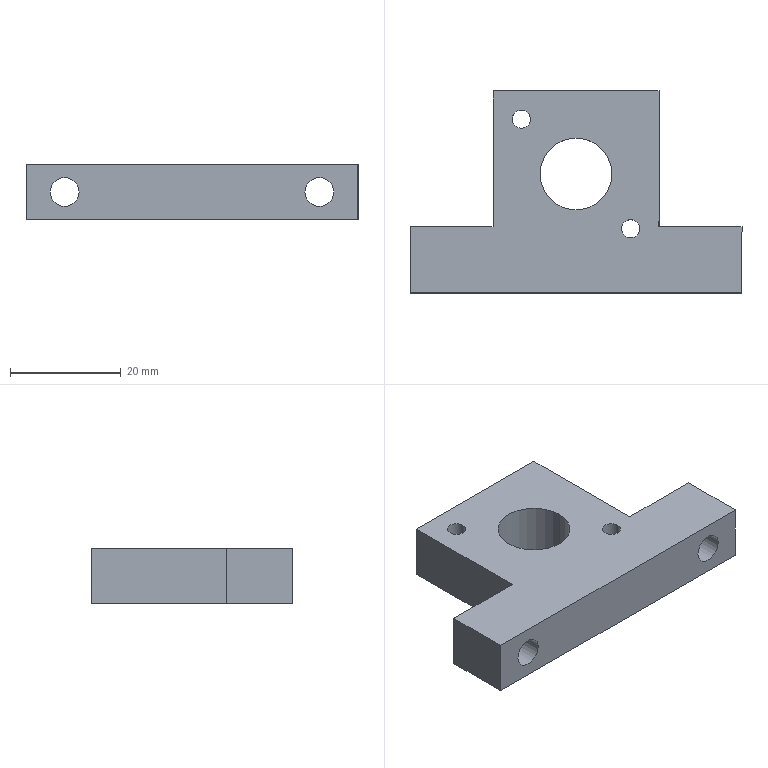Component | SolidWorks | AirCylinderSupportBlock2-1 | 1 solid | 20 faces | box 60 x 36.5 x 10 mm | volume 12542 mm3 | cylinder 10 | plane 10 | commonest cylinder face diameters 3.3 x4 5.2 x4 13 x2 | material 1023 Carbon Steel Plate (SS)
build123d program:
from build123d import *

# Parameters (mm, degrees)
SKETCH1_R                  = 6.5
BOSS_EXTRUDE1_DEPTH        = 10
F_5_2_5_2_DIAMETER_HOLE1_D = 5.2
M4_TAPPED_HOLE1_D          = 3.3
M4_TAPPED_HOLE1_DEPTH      = 11.5
M4_TAPPED_HOLE1_TIP        = 0.9914


with BuildPart() as part:
    # Sketch1 → Boss-Extrude1 (new body)
    with BuildSketch(Plane(origin=(0, 0, 0), x_dir=(0, 0, -1), z_dir=(1, 0, 0))):
        Polygon((73.374, 68.957), (73.374, 44.457), (88.374, 44.457), (88.374, 32.457), (28.374, 32.457), (28.374, 44.457), (43.374, 44.457), (43.374, 68.957), align=None)
        with Locations((58.374, 53.957)):
            Circle(SKETCH1_R, mode=Mode.SUBTRACT)
    extrude(amount=BOSS_EXTRUDE1_DEPTH)

    # 5.2 _5.2_ Diameter Hole1 (through all)
    with Locations(Plane(origin=(0, 44.457, 0), x_dir=(-1, 0, 0), z_dir=(0, 1, 0))):
        with Locations((-5, -35.374), (-5, -81.374)):
            Hole(F_5_2_5_2_DIAMETER_HOLE1_D / 2)

    # M4 Tapped Hole1
    with Locations(Plane(origin=(10, 0, 0), x_dir=(0, 0, -1), z_dir=(1, 0, 0))):
        with Locations((68.274, 63.857), (48.474, 44.057)):
            Hole(M4_TAPPED_HOLE1_D / 2, depth=M4_TAPPED_HOLE1_DEPTH)
            with Locations((0, 0, -(M4_TAPPED_HOLE1_DEPTH + M4_TAPPED_HOLE1_TIP / 2))):  # 118° drill point
                Cone(0, M4_TAPPED_HOLE1_D / 2, M4_TAPPED_HOLE1_TIP, mode=Mode.SUBTRACT)


solid = part.part

# Placed as in the assembly
solid = solid.moved(Location((51.459, -33.763, 34.579), (0, 90, 0)))
STEP:
#1=CARTESIAN_POINT('',(-0.727,1.185,1.361));
#2=VERTEX_POINT('',#1);
#3=CARTESIAN_POINT('',(-0.5971,1.185,1.361));
#4=VERTEX_POINT('',#3);
#5=CARTESIAN_POINT('',(-0.662,1.185,1.361));
#6=DIRECTION('',(-0.,-0.,1.));
#7=DIRECTION('',(1.,-0.,0.));
#8=AXIS2_PLACEMENT_3D('',#5,#6,#7);
#9=CIRCLE('',#8,0.06496);
#10=EDGE_CURVE('',#2,#4,#9,.T.);
#11=ORIENTED_EDGE('',*,*,#10,.T.);
#12=CARTESIAN_POINT('',(-0.5971,1.185,0.9677));
#13=VERTEX_POINT('',#12);
#14=CARTESIAN_POINT('',(-0.5971,1.185,0.9677));
#15=DIRECTION('',(0.,0.,-1.));
#16=VECTOR('',#15,39.37);
#17=LINE('',#14,#16);
#18=EDGE_CURVE('',#4,#13,#17,.T.);
#19=ORIENTED_EDGE('',*,*,#18,.T.);
#20=CARTESIAN_POINT('',(-0.727,1.185,0.9677));
#21=VERTEX_POINT('',#20);
#22=CARTESIAN_POINT('',(-0.662,1.185,0.9677));
#23=DIRECTION('',(0.,0.,-1.));
#24=DIRECTION('',(-1.,0.,0.));
#25=AXIS2_PLACEMENT_3D('',#22,#23,#24);
#26=CIRCLE('',#25,0.06496);
#27=EDGE_CURVE('',#13,#21,#26,.T.);
#28=ORIENTED_EDGE('',*,*,#27,.T.);
#29=CARTESIAN_POINT('',(-0.727,1.185,0.9677));
#30=DIRECTION('',(0.,0.,-1.));
#31=VECTOR('',#30,39.37);
#32=LINE('',#29,#31);
#33=EDGE_CURVE('',#2,#21,#32,.T.);
#34=ORIENTED_EDGE('',*,*,#33,.F.);
#35=EDGE_LOOP('',(#11,#19,#28,#34));
#36=FACE_OUTER_BOUND('',#35,.T.);
#37=CARTESIAN_POINT('',(-0.662,1.185,0.9677));
#38=DIRECTION('',(0.,0.,-1.));
#39=DIRECTION('',(-1.,0.,0.));
#40=AXIS2_PLACEMENT_3D('',#37,#38,#39);
#41=CYLINDRICAL_SURFACE('',#40,0.06496);
#42=ADVANCED_FACE('',(#36),#41,.F.);
#43=CARTESIAN_POINT('',(0.05256,0.4053,1.361));
#44=VERTEX_POINT('',#43);
#45=CARTESIAN_POINT('',(0.1825,0.4053,1.361));
#46=VERTEX_POINT('',#45);
#47=CARTESIAN_POINT('',(0.1175,0.4053,1.361));
#48=DIRECTION('',(-0.,-0.,1.));
#49=DIRECTION('',(1.,-0.,0.));
#50=AXIS2_PLACEMENT_3D('',#47,#48,#49);
#51=CIRCLE('',#50,0.06496);
#52=EDGE_CURVE('',#44,#46,#51,.T.);
#53=ORIENTED_EDGE('',*,*,#52,.T.);
#54=CARTESIAN_POINT('',(0.1825,0.4053,0.9677));
#55=VERTEX_POINT('',#54);
#56=CARTESIAN_POINT('',(0.1825,0.4053,0.9677));
#57=DIRECTION('',(0.,0.,-1.));
#58=VECTOR('',#57,39.37);
#59=LINE('',#56,#58);
#60=EDGE_CURVE('',#46,#55,#59,.T.);
#61=ORIENTED_EDGE('',*,*,#60,.T.);
#62=CARTESIAN_POINT('',(0.05256,0.4053,0.9677));
#63=VERTEX_POINT('',#62);
#64=CARTESIAN_POINT('',(0.1175,0.4053,0.9677));
#65=DIRECTION('',(0.,0.,-1.));
#66=DIRECTION('',(-1.,0.,0.));
#67=AXIS2_PLACEMENT_3D('',#64,#65,#66);
#68=CIRCLE('',#67,0.06496);
#69=EDGE_CURVE('',#55,#63,#68,.T.);
#70=ORIENTED_EDGE('',*,*,#69,.T.);
#71=CARTESIAN_POINT('',(0.05256,0.4053,0.9677));
#72=DIRECTION('',(0.,0.,-1.));
#73=VECTOR('',#72,39.37);
#74=LINE('',#71,#73);
#75=EDGE_CURVE('',#44,#63,#74,.T.);
#76=ORIENTED_EDGE('',*,*,#75,.F.);
#77=EDGE_LOOP('',(#53,#61,#70,#76));
#78=FACE_OUTER_BOUND('',#77,.T.);
#79=CARTESIAN_POINT('',(0.1175,0.4053,0.9677));
#80=DIRECTION('',(0.,0.,-1.));
#81=DIRECTION('',(-1.,0.,0.));
#82=AXIS2_PLACEMENT_3D('',#79,#80,#81);
#83=CYLINDRICAL_SURFACE('',#82,0.06496);
#84=ADVANCED_FACE('',(#78),#83,.F.);
#85=CARTESIAN_POINT('',(0.5309,-0.05139,1.165));
#86=VERTEX_POINT('',#85);
#87=CARTESIAN_POINT('',(0.7356,-0.05139,1.165));
#88=VERTEX_POINT('',#87);
#89=CARTESIAN_POINT('',(0.6333,-0.05139,1.165));
#90=DIRECTION('',(0.,1.,0.));
#91=DIRECTION('',(1.,-0.,0.));
#92=AXIS2_PLACEMENT_3D('',#89,#90,#91);
#93=CIRCLE('',#92,0.1024);
#94=EDGE_CURVE('',#86,#88,#93,.T.);
#95=ORIENTED_EDGE('',*,*,#94,.F.);
#96=CARTESIAN_POINT('',(0.5309,0.421,1.165));
#97=VERTEX_POINT('',#96);
#98=CARTESIAN_POINT('',(0.5309,0.421,1.165));
#99=DIRECTION('',(0.,1.,0.));
#100=VECTOR('',#99,39.37);
#101=LINE('',#98,#100);
#102=EDGE_CURVE('',#86,#97,#101,.T.);
#103=ORIENTED_EDGE('',*,*,#102,.T.);
#104=CARTESIAN_POINT('',(0.7356,0.421,1.165));
#105=VERTEX_POINT('',#104);
#106=CARTESIAN_POINT('',(0.6333,0.421,1.165));
#107=DIRECTION('',(0.,1.,0.));
#108=DIRECTION('',(1.,-0.,0.));
#109=AXIS2_PLACEMENT_3D('',#106,#107,#108);
#110=CIRCLE('',#109,0.1024);
#111=EDGE_CURVE('',#97,#105,#110,.T.);
#112=ORIENTED_EDGE('',*,*,#111,.T.);
#113=CARTESIAN_POINT('',(0.7356,0.421,1.165));
#114=DIRECTION('',(0.,1.,0.));
#115=VECTOR('',#114,39.37);
#116=LINE('',#113,#115);
#117=EDGE_CURVE('',#88,#105,#116,.T.);
#118=ORIENTED_EDGE('',*,*,#117,.F.);
#119=EDGE_LOOP('',(#95,#103,#112,#118));
#120=FACE_OUTER_BOUND('',#119,.T.);
#121=CARTESIAN_POINT('',(0.6333,0.421,1.165));
#122=DIRECTION('',(0.,1.,0.));
#123=DIRECTION('',(1.,-0.,0.));
#124=AXIS2_PLACEMENT_3D('',#121,#122,#123);
#125=CYLINDRICAL_SURFACE('',#124,0.1024);
#126=ADVANCED_FACE('',(#120),#125,.F.);
#127=CARTESIAN_POINT('',(-1.28,-0.05139,1.165));
#128=VERTEX_POINT('',#127);
#129=CARTESIAN_POINT('',(-1.075,-0.05139,1.165));
#130=VERTEX_POINT('',#129);
#131=CARTESIAN_POINT('',(-1.178,-0.05139,1.165));
#132=DIRECTION('',(0.,1.,0.));
#133=DIRECTION('',(1.,-0.,0.));
#134=AXIS2_PLACEMENT_3D('',#131,#132,#133);
#135=CIRCLE('',#134,0.1024);
#136=EDGE_CURVE('',#128,#130,#135,.T.);
#137=ORIENTED_EDGE('',*,*,#136,.F.);
#138=CARTESIAN_POINT('',(-1.28,0.421,1.165));
#139=VERTEX_POINT('',#138);
#140=CARTESIAN_POINT('',(-1.28,0.421,1.165));
#141=DIRECTION('',(0.,1.,0.));
#142=VECTOR('',#141,39.37);
#143=LINE('',#140,#142);
#144=EDGE_CURVE('',#128,#139,#143,.T.);
#145=ORIENTED_EDGE('',*,*,#144,.T.);
#146=CARTESIAN_POINT('',(-1.075,0.421,1.165));
#147=VERTEX_POINT('',#146);
#148=CARTESIAN_POINT('',(-1.178,0.421,1.165));
#149=DIRECTION('',(0.,1.,0.));
#150=DIRECTION('',(1.,-0.,0.));
#151=AXIS2_PLACEMENT_3D('',#148,#149,#150);
#152=CIRCLE('',#151,0.1024);
#153=EDGE_CURVE('',#139,#147,#152,.T.);
#154=ORIENTED_EDGE('',*,*,#153,.T.);
#155=CARTESIAN_POINT('',(-1.075,0.421,1.165));
#156=DIRECTION('',(0.,1.,0.));
#157=VECTOR('',#156,39.37);
#158=LINE('',#155,#157);
#159=EDGE_CURVE('',#130,#147,#158,.T.);
#160=ORIENTED_EDGE('',*,*,#159,.F.);
#161=EDGE_LOOP('',(#137,#145,#154,#160));
#162=FACE_OUTER_BOUND('',#161,.T.);
#163=CARTESIAN_POINT('',(-1.178,0.421,1.165));
#164=DIRECTION('',(0.,1.,0.));
#165=DIRECTION('',(1.,-0.,0.));
#166=AXIS2_PLACEMENT_3D('',#163,#164,#165);
#167=CYLINDRICAL_SURFACE('',#166,0.1024);
#168=ADVANCED_FACE('',(#162),#167,.F.);
#169=CARTESIAN_POINT('',(-0.01634,0.7951,0.9677));
#170=VERTEX_POINT('',#169);
#171=CARTESIAN_POINT('',(-0.5282,0.7951,0.9677));
#172=VERTEX_POINT('',#171);
#173=CARTESIAN_POINT('',(-0.2722,0.7951,0.9677));
#174=DIRECTION('',(0.,0.,-1.));
#175=DIRECTION('',(-1.,0.,0.));
#176=AXIS2_PLACEMENT_3D('',#173,#174,#175);
#177=CIRCLE('',#176,0.2559);
#178=EDGE_CURVE('',#170,#172,#177,.T.);
#179=ORIENTED_EDGE('',*,*,#178,.T.);
#180=CARTESIAN_POINT('',(-0.5282,0.7951,1.361));
#181=VERTEX_POINT('',#180);
#182=CARTESIAN_POINT('',(-0.5282,0.7951,0.9677));
#183=DIRECTION('',(-0.,-0.,1.));
#184=VECTOR('',#183,39.37);
#185=LINE('',#182,#184);
#186=EDGE_CURVE('',#172,#181,#185,.T.);
#187=ORIENTED_EDGE('',*,*,#186,.T.);
#188=CARTESIAN_POINT('',(-0.01634,0.7951,1.361));
#189=VERTEX_POINT('',#188);
#190=CARTESIAN_POINT('',(-0.2722,0.7951,1.361));
#191=DIRECTION('',(0.,0.,-1.));
#192=DIRECTION('',(-1.,0.,0.));
#193=AXIS2_PLACEMENT_3D('',#190,#191,#192);
#194=CIRCLE('',#193,0.2559);
#195=EDGE_CURVE('',#189,#181,#194,.T.);
#196=ORIENTED_EDGE('',*,*,#195,.F.);
#197=CARTESIAN_POINT('',(-0.01634,0.7951,0.9677));
#198=DIRECTION('',(-0.,-0.,1.));
#199=VECTOR('',#198,39.37);
#200=LINE('',#197,#199);
#201=EDGE_CURVE('',#170,#189,#200,.T.);
#202=ORIENTED_EDGE('',*,*,#201,.F.);
#203=EDGE_LOOP('',(#179,#187,#196,#202));
#204=FACE_OUTER_BOUND('',#203,.T.);
#205=CARTESIAN_POINT('',(-0.2722,0.7951,0.9677));
#206=DIRECTION('',(-0.,-0.,1.));
#207=DIRECTION('',(1.,-0.,0.));
#208=AXIS2_PLACEMENT_3D('',#205,#206,#207);
#209=CYLINDRICAL_SURFACE('',#208,0.2559);
#210=ADVANCED_FACE('',(#204),#209,.F.);
#211=CARTESIAN_POINT('',(-0.662,1.185,0.9677));
#212=DIRECTION('',(0.,0.,-1.));
#213=DIRECTION('',(-1.,0.,0.));
#214=AXIS2_PLACEMENT_3D('',#211,#212,#213);
#215=CIRCLE('',#214,0.06496);
#216=EDGE_CURVE('',#21,#13,#215,.T.);
#217=ORIENTED_EDGE('',*,*,#216,.F.);
#218=ORIENTED_EDGE('',*,*,#27,.F.);
#219=EDGE_LOOP('',(#217,#218));
#220=FACE_BOUND('',#219,.T.);
#221=CARTESIAN_POINT('',(0.1175,0.4053,0.9677));
#222=DIRECTION('',(0.,0.,-1.));
#223=DIRECTION('',(-1.,0.,0.));
#224=AXIS2_PLACEMENT_3D('',#221,#222,#223);
#225=CIRCLE('',#224,0.06496);
#226=EDGE_CURVE('',#63,#55,#225,.T.);
#227=ORIENTED_EDGE('',*,*,#226,.F.);
#228=ORIENTED_EDGE('',*,*,#69,.F.);
#229=EDGE_LOOP('',(#227,#228));
#230=FACE_BOUND('',#229,.T.);
#231=CARTESIAN_POINT('',(-0.8628,1.386,0.9677));
#232=VERTEX_POINT('',#231);
#233=CARTESIAN_POINT('',(0.3183,1.386,0.9677));
#234=VERTEX_POINT('',#233);
#235=CARTESIAN_POINT('',(0.3183,1.386,0.9677));
#236=DIRECTION('',(1.,-0.,0.));
#237=VECTOR('',#236,39.37);
#238=LINE('',#235,#237);
#239=EDGE_CURVE('',#232,#234,#238,.T.);
#240=ORIENTED_EDGE('',*,*,#239,.T.);
#241=CARTESIAN_POINT('',(0.3183,0.421,0.9677));
#242=VERTEX_POINT('',#241);
#243=CARTESIAN_POINT('',(0.3183,1.386,0.9677));
#244=DIRECTION('',(-0.,-1.,-0.));
#245=VECTOR('',#244,39.37);
#246=LINE('',#243,#245);
#247=EDGE_CURVE('',#234,#242,#246,.T.);
#248=ORIENTED_EDGE('',*,*,#247,.T.);
#249=CARTESIAN_POINT('',(0.9089,0.421,0.9677));
#250=VERTEX_POINT('',#249);
#251=CARTESIAN_POINT('',(0.9089,0.421,0.9677));
#252=DIRECTION('',(1.,-0.,0.));
#253=VECTOR('',#252,39.37);
#254=LINE('',#251,#253);
#255=EDGE_CURVE('',#242,#250,#254,.T.);
#256=ORIENTED_EDGE('',*,*,#255,.T.);
#257=CARTESIAN_POINT('',(0.9089,-0.05139,0.9677));
#258=VERTEX_POINT('',#257);
#259=CARTESIAN_POINT('',(0.9089,-0.05139,0.9677));
#260=DIRECTION('',(-0.,-1.,-0.));
#261=VECTOR('',#260,39.37);
#262=LINE('',#259,#261);
#263=EDGE_CURVE('',#250,#258,#262,.T.);
#264=ORIENTED_EDGE('',*,*,#263,.T.);
#265=CARTESIAN_POINT('',(-1.453,-0.05139,0.9677));
#266=VERTEX_POINT('',#265);
#267=CARTESIAN_POINT('',(-1.453,-0.05139,0.9677));
#268=DIRECTION('',(-1.,0.,-0.));
#269=VECTOR('',#268,39.37);
#270=LINE('',#267,#269);
#271=EDGE_CURVE('',#258,#266,#270,.T.);
#272=ORIENTED_EDGE('',*,*,#271,.T.);
#273=CARTESIAN_POINT('',(-1.453,0.421,0.9677));
#274=VERTEX_POINT('',#273);
#275=CARTESIAN_POINT('',(-1.453,0.421,0.9677));
#276=DIRECTION('',(0.,1.,0.));
#277=VECTOR('',#276,39.37);
#278=LINE('',#275,#277);
#279=EDGE_CURVE('',#266,#274,#278,.T.);
#280=ORIENTED_EDGE('',*,*,#279,.T.);
#281=CARTESIAN_POINT('',(-0.8628,0.421,0.9677));
#282=VERTEX_POINT('',#281);
#283=CARTESIAN_POINT('',(-0.8628,0.421,0.9677));
#284=DIRECTION('',(1.,-0.,0.));
#285=VECTOR('',#284,39.37);
#286=LINE('',#283,#285);
#287=EDGE_CURVE('',#274,#282,#286,.T.);
#288=ORIENTED_EDGE('',*,*,#287,.T.);
#289=CARTESIAN_POINT('',(-0.8628,1.386,0.9677));
#290=DIRECTION('',(0.,1.,0.));
#291=VECTOR('',#290,39.37);
#292=LINE('',#289,#291);
#293=EDGE_CURVE('',#282,#232,#292,.T.);
#294=ORIENTED_EDGE('',*,*,#293,.T.);
#295=EDGE_LOOP('',(#240,#248,#256,#264,#272,#280,#288,#294));
#296=FACE_OUTER_BOUND('',#295,.T.);
#297=ORIENTED_EDGE('',*,*,#178,.F.);
#298=CARTESIAN_POINT('',(-0.2722,0.7951,0.9677));
#299=DIRECTION('',(0.,0.,-1.));
#300=DIRECTION('',(-1.,0.,0.));
#301=AXIS2_PLACEMENT_3D('',#298,#299,#300);
#302=CIRCLE('',#301,0.2559);
#303=EDGE_CURVE('',#172,#170,#302,.T.);
#304=ORIENTED_EDGE('',*,*,#303,.F.);
#305=EDGE_LOOP('',(#297,#304));
#306=FACE_BOUND('',#305,.T.);
#307=CARTESIAN_POINT('',(-0.8628,1.386,0.9677));
#308=DIRECTION('',(-0.,-0.,1.));
#309=DIRECTION('',(1.,-0.,0.));
#310=AXIS2_PLACEMENT_3D('',#307,#308,#309);
#311=PLANE('',#310);
#312=ADVANCED_FACE('',(#220,#230,#296,#306),#311,.F.);
#313=ORIENTED_EDGE('',*,*,#10,.F.);
#314=CARTESIAN_POINT('',(-0.662,1.185,1.361));
#315=DIRECTION('',(-0.,-0.,1.));
#316=DIRECTION('',(1.,-0.,0.));
#317=AXIS2_PLACEMENT_3D('',#314,#315,#316);
#318=CIRCLE('',#317,0.06496);
#319=EDGE_CURVE('',#4,#2,#318,.T.);
#320=ORIENTED_EDGE('',*,*,#319,.F.);
#321=EDGE_LOOP('',(#313,#320));
#322=FACE_BOUND('',#321,.T.);
#323=ORIENTED_EDGE('',*,*,#52,.F.);
#324=CARTESIAN_POINT('',(0.1175,0.4053,1.361));
#325=DIRECTION('',(-0.,-0.,1.));
#326=DIRECTION('',(1.,-0.,0.));
#327=AXIS2_PLACEMENT_3D('',#324,#325,#326);
#328=CIRCLE('',#327,0.06496);
#329=EDGE_CURVE('',#46,#44,#328,.T.);
#330=ORIENTED_EDGE('',*,*,#329,.F.);
#331=EDGE_LOOP('',(#323,#330));
#332=FACE_BOUND('',#331,.T.);
#333=CARTESIAN_POINT('',(-0.8628,1.386,1.361));
#334=VERTEX_POINT('',#333);
#335=CARTESIAN_POINT('',(0.3183,1.386,1.361));
#336=VERTEX_POINT('',#335);
#337=CARTESIAN_POINT('',(0.3183,1.386,1.361));
#338=DIRECTION('',(1.,-0.,0.));
#339=VECTOR('',#338,39.37);
#340=LINE('',#337,#339);
#341=EDGE_CURVE('',#334,#336,#340,.T.);
#342=ORIENTED_EDGE('',*,*,#341,.F.);
#343=CARTESIAN_POINT('',(-0.8628,0.421,1.361));
#344=VERTEX_POINT('',#343);
#345=CARTESIAN_POINT('',(-0.8628,1.386,1.361));
#346=DIRECTION('',(0.,1.,0.));
#347=VECTOR('',#346,39.37);
#348=LINE('',#345,#347);
#349=EDGE_CURVE('',#344,#334,#348,.T.);
#350=ORIENTED_EDGE('',*,*,#349,.F.);
#351=CARTESIAN_POINT('',(-1.453,0.421,1.361));
#352=VERTEX_POINT('',#351);
#353=CARTESIAN_POINT('',(-0.8628,0.421,1.361));
#354=DIRECTION('',(1.,-0.,0.));
#355=VECTOR('',#354,39.37);
#356=LINE('',#353,#355);
#357=EDGE_CURVE('',#352,#344,#356,.T.);
#358=ORIENTED_EDGE('',*,*,#357,.F.);
#359=CARTESIAN_POINT('',(-1.453,-0.05139,1.361));
#360=VERTEX_POINT('',#359);
#361=CARTESIAN_POINT('',(-1.453,0.421,1.361));
#362=DIRECTION('',(0.,1.,0.));
#363=VECTOR('',#362,39.37);
#364=LINE('',#361,#363);
#365=EDGE_CURVE('',#360,#352,#364,.T.);
#366=ORIENTED_EDGE('',*,*,#365,.F.);
#367=CARTESIAN_POINT('',(0.9089,-0.05139,1.361));
#368=VERTEX_POINT('',#367);
#369=CARTESIAN_POINT('',(-1.453,-0.05139,1.361));
#370=DIRECTION('',(-1.,0.,-0.));
#371=VECTOR('',#370,39.37);
#372=LINE('',#369,#371);
#373=EDGE_CURVE('',#368,#360,#372,.T.);
#374=ORIENTED_EDGE('',*,*,#373,.F.);
#375=CARTESIAN_POINT('',(0.9089,0.421,1.361));
#376=VERTEX_POINT('',#375);
#377=CARTESIAN_POINT('',(0.9089,-0.05139,1.361));
#378=DIRECTION('',(-0.,-1.,-0.));
#379=VECTOR('',#378,39.37);
#380=LINE('',#377,#379);
#381=EDGE_CURVE('',#376,#368,#380,.T.);
#382=ORIENTED_EDGE('',*,*,#381,.F.);
#383=CARTESIAN_POINT('',(0.3183,0.421,1.361));
#384=VERTEX_POINT('',#383);
#385=CARTESIAN_POINT('',(0.9089,0.421,1.361));
#386=DIRECTION('',(1.,-0.,0.));
#387=VECTOR('',#386,39.37);
#388=LINE('',#385,#387);
#389=EDGE_CURVE('',#384,#376,#388,.T.);
#390=ORIENTED_EDGE('',*,*,#389,.F.);
#391=CARTESIAN_POINT('',(0.3183,1.386,1.361));
#392=DIRECTION('',(-0.,-1.,-0.));
#393=VECTOR('',#392,39.37);
#394=LINE('',#391,#393);
#395=EDGE_CURVE('',#336,#384,#394,.T.);
#396=ORIENTED_EDGE('',*,*,#395,.F.);
#397=EDGE_LOOP('',(#342,#350,#358,#366,#374,#382,#390,#396));
#398=FACE_OUTER_BOUND('',#397,.T.);
#399=ORIENTED_EDGE('',*,*,#195,.T.);
#400=CARTESIAN_POINT('',(-0.2722,0.7951,1.361));
#401=DIRECTION('',(0.,0.,-1.));
#402=DIRECTION('',(-1.,0.,0.));
#403=AXIS2_PLACEMENT_3D('',#400,#401,#402);
#404=CIRCLE('',#403,0.2559);
#405=EDGE_CURVE('',#181,#189,#404,.T.);
#406=ORIENTED_EDGE('',*,*,#405,.T.);
#407=EDGE_LOOP('',(#399,#406));
#408=FACE_BOUND('',#407,.T.);
#409=CARTESIAN_POINT('',(-0.8628,1.386,1.361));
#410=DIRECTION('',(-0.,-0.,1.));
#411=DIRECTION('',(1.,-0.,0.));
#412=AXIS2_PLACEMENT_3D('',#409,#410,#411);
#413=PLANE('',#412);
#414=ADVANCED_FACE('',(#322,#332,#398,#408),#413,.T.);
#415=ORIENTED_EDGE('',*,*,#341,.T.);
#416=CARTESIAN_POINT('',(0.3183,1.386,0.9677));
#417=DIRECTION('',(-0.,-0.,1.));
#418=VECTOR('',#417,39.37);
#419=LINE('',#416,#418);
#420=EDGE_CURVE('',#234,#336,#419,.T.);
#421=ORIENTED_EDGE('',*,*,#420,.F.);
#422=ORIENTED_EDGE('',*,*,#239,.F.);
#423=CARTESIAN_POINT('',(-0.8628,1.386,0.9677));
#424=DIRECTION('',(-0.,-0.,1.));
#425=VECTOR('',#424,39.37);
#426=LINE('',#423,#425);
#427=EDGE_CURVE('',#232,#334,#426,.T.);
#428=ORIENTED_EDGE('',*,*,#427,.T.);
#429=EDGE_LOOP('',(#415,#421,#422,#428));
#430=FACE_OUTER_BOUND('',#429,.T.);
#431=CARTESIAN_POINT('',(0.3183,1.386,0.9677));
#432=DIRECTION('',(-0.,-1.,-0.));
#433=DIRECTION('',(-1.,0.,-0.));
#434=AXIS2_PLACEMENT_3D('',#431,#432,#433);
#435=PLANE('',#434);
#436=ADVANCED_FACE('',(#430),#435,.F.);
#437=ORIENTED_EDGE('',*,*,#395,.T.);
#438=CARTESIAN_POINT('',(0.3183,0.421,0.9677));
#439=DIRECTION('',(-0.,-0.,1.));
#440=VECTOR('',#439,39.37);
#441=LINE('',#438,#440);
#442=EDGE_CURVE('',#242,#384,#441,.T.);
#443=ORIENTED_EDGE('',*,*,#442,.F.);
#444=ORIENTED_EDGE('',*,*,#247,.F.);
#445=ORIENTED_EDGE('',*,*,#420,.T.);
#446=EDGE_LOOP('',(#437,#443,#444,#445));
#447=FACE_OUTER_BOUND('',#446,.T.);
#448=CARTESIAN_POINT('',(0.3183,1.386,0.9677));
#449=DIRECTION('',(-1.,0.,-0.));
#450=DIRECTION('',(0.,1.,0.));
#451=AXIS2_PLACEMENT_3D('',#448,#449,#450);
#452=PLANE('',#451);
#453=ADVANCED_FACE('',(#447),#452,.F.);
#454=CARTESIAN_POINT('',(0.6333,0.421,1.165));
#455=DIRECTION('',(0.,1.,0.));
#456=DIRECTION('',(1.,-0.,0.));
#457=AXIS2_PLACEMENT_3D('',#454,#455,#456);
#458=CIRCLE('',#457,0.1024);
#459=EDGE_CURVE('',#105,#97,#458,.T.);
#460=ORIENTED_EDGE('',*,*,#459,.F.);
#461=ORIENTED_EDGE('',*,*,#111,.F.);
#462=EDGE_LOOP('',(#460,#461));
#463=FACE_BOUND('',#462,.T.);
#464=ORIENTED_EDGE('',*,*,#389,.T.);
#465=CARTESIAN_POINT('',(0.9089,0.421,0.9677));
#466=DIRECTION('',(-0.,-0.,1.));
#467=VECTOR('',#466,39.37);
#468=LINE('',#465,#467);
#469=EDGE_CURVE('',#250,#376,#468,.T.);
#470=ORIENTED_EDGE('',*,*,#469,.F.);
#471=ORIENTED_EDGE('',*,*,#255,.F.);
#472=ORIENTED_EDGE('',*,*,#442,.T.);
#473=EDGE_LOOP('',(#464,#470,#471,#472));
#474=FACE_OUTER_BOUND('',#473,.T.);
#475=CARTESIAN_POINT('',(0.9089,0.421,0.9677));
#476=DIRECTION('',(-0.,-1.,-0.));
#477=DIRECTION('',(-1.,0.,-0.));
#478=AXIS2_PLACEMENT_3D('',#475,#476,#477);
#479=PLANE('',#478);
#480=ADVANCED_FACE('',(#463,#474),#479,.F.);
#481=ORIENTED_EDGE('',*,*,#381,.T.);
#482=CARTESIAN_POINT('',(0.9089,-0.05139,0.9677));
#483=DIRECTION('',(-0.,-0.,1.));
#484=VECTOR('',#483,39.37);
#485=LINE('',#482,#484);
#486=EDGE_CURVE('',#258,#368,#485,.T.);
#487=ORIENTED_EDGE('',*,*,#486,.F.);
#488=ORIENTED_EDGE('',*,*,#263,.F.);
#489=ORIENTED_EDGE('',*,*,#469,.T.);
#490=EDGE_LOOP('',(#481,#487,#488,#489));
#491=FACE_OUTER_BOUND('',#490,.T.);
#492=CARTESIAN_POINT('',(0.9089,-0.05139,0.9677));
#493=DIRECTION('',(-1.,0.,-0.));
#494=DIRECTION('',(-0.,-0.,1.));
#495=AXIS2_PLACEMENT_3D('',#492,#493,#494);
#496=PLANE('',#495);
#497=ADVANCED_FACE('',(#491),#496,.F.);
#498=CARTESIAN_POINT('',(0.6333,-0.05139,1.165));
#499=DIRECTION('',(0.,1.,0.));
#500=DIRECTION('',(1.,-0.,0.));
#501=AXIS2_PLACEMENT_3D('',#498,#499,#500);
#502=CIRCLE('',#501,0.1024);
#503=EDGE_CURVE('',#88,#86,#502,.T.);
#504=ORIENTED_EDGE('',*,*,#503,.T.);
#505=ORIENTED_EDGE('',*,*,#94,.T.);
#506=EDGE_LOOP('',(#504,#505));
#507=FACE_BOUND('',#506,.T.);
#508=CARTESIAN_POINT('',(-1.178,-0.05139,1.165));
#509=DIRECTION('',(0.,1.,0.));
#510=DIRECTION('',(1.,-0.,0.));
#511=AXIS2_PLACEMENT_3D('',#508,#509,#510);
#512=CIRCLE('',#511,0.1024);
#513=EDGE_CURVE('',#130,#128,#512,.T.);
#514=ORIENTED_EDGE('',*,*,#513,.T.);
#515=ORIENTED_EDGE('',*,*,#136,.T.);
#516=EDGE_LOOP('',(#514,#515));
#517=FACE_BOUND('',#516,.T.);
#518=ORIENTED_EDGE('',*,*,#373,.T.);
#519=CARTESIAN_POINT('',(-1.453,-0.05139,0.9677));
#520=DIRECTION('',(-0.,-0.,1.));
#521=VECTOR('',#520,39.37);
#522=LINE('',#519,#521);
#523=EDGE_CURVE('',#266,#360,#522,.T.);
#524=ORIENTED_EDGE('',*,*,#523,.F.);
#525=ORIENTED_EDGE('',*,*,#271,.F.);
#526=ORIENTED_EDGE('',*,*,#486,.T.);
#527=EDGE_LOOP('',(#518,#524,#525,#526));
#528=FACE_OUTER_BOUND('',#527,.T.);
#529=CARTESIAN_POINT('',(-1.453,-0.05139,0.9677));
#530=DIRECTION('',(0.,1.,0.));
#531=DIRECTION('',(1.,-0.,0.));
#532=AXIS2_PLACEMENT_3D('',#529,#530,#531);
#533=PLANE('',#532);
#534=ADVANCED_FACE('',(#507,#517,#528),#533,.F.);
#535=ORIENTED_EDGE('',*,*,#365,.T.);
#536=CARTESIAN_POINT('',(-1.453,0.421,0.9677));
#537=DIRECTION('',(-0.,-0.,1.));
#538=VECTOR('',#537,39.37);
#539=LINE('',#536,#538);
#540=EDGE_CURVE('',#274,#352,#539,.T.);
#541=ORIENTED_EDGE('',*,*,#540,.F.);
#542=ORIENTED_EDGE('',*,*,#279,.F.);
#543=ORIENTED_EDGE('',*,*,#523,.T.);
#544=EDGE_LOOP('',(#535,#541,#542,#543));
#545=FACE_OUTER_BOUND('',#544,.T.);
#546=CARTESIAN_POINT('',(-1.453,0.421,0.9677));
#547=DIRECTION('',(1.,-0.,0.));
#548=DIRECTION('',(-0.,-1.,-0.));
#549=AXIS2_PLACEMENT_3D('',#546,#547,#548);
#550=PLANE('',#549);
#551=ADVANCED_FACE('',(#545),#550,.F.);
#552=CARTESIAN_POINT('',(-1.178,0.421,1.165));
#553=DIRECTION('',(0.,1.,0.));
#554=DIRECTION('',(1.,-0.,0.));
#555=AXIS2_PLACEMENT_3D('',#552,#553,#554);
#556=CIRCLE('',#555,0.1024);
#557=EDGE_CURVE('',#147,#139,#556,.T.);
#558=ORIENTED_EDGE('',*,*,#557,.F.);
#559=ORIENTED_EDGE('',*,*,#153,.F.);
#560=EDGE_LOOP('',(#558,#559));
#561=FACE_BOUND('',#560,.T.);
#562=ORIENTED_EDGE('',*,*,#357,.T.);
#563=CARTESIAN_POINT('',(-0.8628,0.421,0.9677));
#564=DIRECTION('',(-0.,-0.,1.));
#565=VECTOR('',#564,39.37);
#566=LINE('',#563,#565);
#567=EDGE_CURVE('',#282,#344,#566,.T.);
#568=ORIENTED_EDGE('',*,*,#567,.F.);
#569=ORIENTED_EDGE('',*,*,#287,.F.);
#570=ORIENTED_EDGE('',*,*,#540,.T.);
#571=EDGE_LOOP('',(#562,#568,#569,#570));
#572=FACE_OUTER_BOUND('',#571,.T.);
#573=CARTESIAN_POINT('',(-0.8628,0.421,0.9677));
#574=DIRECTION('',(-0.,-1.,-0.));
#575=DIRECTION('',(-1.,0.,-0.));
#576=AXIS2_PLACEMENT_3D('',#573,#574,#575);
#577=PLANE('',#576);
#578=ADVANCED_FACE('',(#561,#572),#577,.F.);
#579=ORIENTED_EDGE('',*,*,#349,.T.);
#580=ORIENTED_EDGE('',*,*,#427,.F.);
#581=ORIENTED_EDGE('',*,*,#293,.F.);
#582=ORIENTED_EDGE('',*,*,#567,.T.);
#583=EDGE_LOOP('',(#579,#580,#581,#582));
#584=FACE_OUTER_BOUND('',#583,.T.);
#585=CARTESIAN_POINT('',(-0.8628,1.386,0.9677));
#586=DIRECTION('',(1.,-0.,0.));
#587=DIRECTION('',(-0.,-1.,-0.));
#588=AXIS2_PLACEMENT_3D('',#585,#586,#587);
#589=PLANE('',#588);
#590=ADVANCED_FACE('',(#584),#589,.F.);
#591=ORIENTED_EDGE('',*,*,#186,.F.);
#592=ORIENTED_EDGE('',*,*,#303,.T.);
#593=ORIENTED_EDGE('',*,*,#201,.T.);
#594=ORIENTED_EDGE('',*,*,#405,.F.);
#595=EDGE_LOOP('',(#591,#592,#593,#594));
#596=FACE_OUTER_BOUND('',#595,.T.);
#597=CARTESIAN_POINT('',(-0.2722,0.7951,0.9677));
#598=DIRECTION('',(-0.,-0.,1.));
#599=DIRECTION('',(1.,-0.,0.));
#600=AXIS2_PLACEMENT_3D('',#597,#598,#599);
#601=CYLINDRICAL_SURFACE('',#600,0.2559);
#602=ADVANCED_FACE('',(#596),#601,.F.);
#603=ORIENTED_EDGE('',*,*,#144,.F.);
#604=ORIENTED_EDGE('',*,*,#513,.F.);
#605=ORIENTED_EDGE('',*,*,#159,.T.);
#606=ORIENTED_EDGE('',*,*,#557,.T.);
#607=EDGE_LOOP('',(#603,#604,#605,#606));
#608=FACE_OUTER_BOUND('',#607,.T.);
#609=CARTESIAN_POINT('',(-1.178,0.421,1.165));
#610=DIRECTION('',(0.,1.,0.));
#611=DIRECTION('',(1.,-0.,0.));
#612=AXIS2_PLACEMENT_3D('',#609,#610,#611);
#613=CYLINDRICAL_SURFACE('',#612,0.1024);
#614=ADVANCED_FACE('',(#608),#613,.F.);
#615=ORIENTED_EDGE('',*,*,#102,.F.);
#616=ORIENTED_EDGE('',*,*,#503,.F.);
#617=ORIENTED_EDGE('',*,*,#117,.T.);
#618=ORIENTED_EDGE('',*,*,#459,.T.);
#619=EDGE_LOOP('',(#615,#616,#617,#618));
#620=FACE_OUTER_BOUND('',#619,.T.);
#621=CARTESIAN_POINT('',(0.6333,0.421,1.165));
#622=DIRECTION('',(0.,1.,0.));
#623=DIRECTION('',(1.,-0.,0.));
#624=AXIS2_PLACEMENT_3D('',#621,#622,#623);
#625=CYLINDRICAL_SURFACE('',#624,0.1024);
#626=ADVANCED_FACE('',(#620),#625,.F.);
#627=ORIENTED_EDGE('',*,*,#60,.F.);
#628=ORIENTED_EDGE('',*,*,#329,.T.);
#629=ORIENTED_EDGE('',*,*,#75,.T.);
#630=ORIENTED_EDGE('',*,*,#226,.T.);
#631=EDGE_LOOP('',(#627,#628,#629,#630));
#632=FACE_OUTER_BOUND('',#631,.T.);
#633=CARTESIAN_POINT('',(0.1175,0.4053,0.9677));
#634=DIRECTION('',(0.,0.,-1.));
#635=DIRECTION('',(-1.,0.,0.));
#636=AXIS2_PLACEMENT_3D('',#633,#634,#635);
#637=CYLINDRICAL_SURFACE('',#636,0.06496);
#638=ADVANCED_FACE('',(#632),#637,.F.);
#639=ORIENTED_EDGE('',*,*,#18,.F.);
#640=ORIENTED_EDGE('',*,*,#319,.T.);
#641=ORIENTED_EDGE('',*,*,#33,.T.);
#642=ORIENTED_EDGE('',*,*,#216,.T.);
#643=EDGE_LOOP('',(#639,#640,#641,#642));
#644=FACE_OUTER_BOUND('',#643,.T.);
#645=CARTESIAN_POINT('',(-0.662,1.185,0.9677));
#646=DIRECTION('',(0.,0.,-1.));
#647=DIRECTION('',(-1.,0.,0.));
#648=AXIS2_PLACEMENT_3D('',#645,#646,#647);
#649=CYLINDRICAL_SURFACE('',#648,0.06496);
#650=ADVANCED_FACE('',(#644),#649,.F.);
#651=CLOSED_SHELL('',(#42,#84,#126,#168,#210,#312,#414,#436,#453,#480,#497,#534,#551,#578,#590,#602,#614,#626,#638,#650));
#652=MANIFOLD_SOLID_BREP('',#651);
#653=CARTESIAN_POINT('',(0.,0.,0.));
#654=DIRECTION('',(0.,0.,1.));
#655=DIRECTION('',(1.,0.,0.));
#656=AXIS2_PLACEMENT_3D('',#653,#654,#655);
#657=(LENGTH_UNIT()NAMED_UNIT(*)SI_UNIT($,.METRE.));
#658=LENGTH_MEASURE_WITH_UNIT(LENGTH_MEASURE(0.0254),#657);
#659=DIMENSIONAL_EXPONENTS(1.,0.,0.,0.,0.,0.,0.);
#660=(CONVERSION_BASED_UNIT('',#658)LENGTH_UNIT()NAMED_UNIT(#659));
#661=UNCERTAINTY_MEASURE_WITH_UNIT(LENGTH_MEASURE(0.00001),#660,'','');
#662=(NAMED_UNIT(*)PLANE_ANGLE_UNIT()SI_UNIT($,.RADIAN.));
#663=(NAMED_UNIT(*)SI_UNIT($,.STERADIAN.)SOLID_ANGLE_UNIT());
#664=(GEOMETRIC_REPRESENTATION_CONTEXT(3)GLOBAL_UNCERTAINTY_ASSIGNED_CONTEXT((#661))GLOBAL_UNIT_ASSIGNED_CONTEXT((#660,#662,#663))REPRESENTATION_CONTEXT('',''));
#665=ADVANCED_BREP_SHAPE_REPRESENTATION('',(#652,#656),#664);
#666=COLOUR_RGB('',0.7922,0.8196,0.9333);
#667=FILL_AREA_STYLE_COLOUR('',#666);
#668=FILL_AREA_STYLE('',(#667));
#669=SURFACE_STYLE_FILL_AREA(#668);
#670=SURFACE_SIDE_STYLE('',(#669));
#671=SURFACE_STYLE_USAGE(.BOTH.,#670);
#672=PRESENTATION_STYLE_ASSIGNMENT((#671));
#673=STYLED_ITEM('',(#672),#652);
#674=PRESENTATION_LAYER_ASSIGNMENT('','',(#673));
#675=(LENGTH_UNIT()NAMED_UNIT(*)SI_UNIT($,.METRE.));
#676=LENGTH_MEASURE_WITH_UNIT(LENGTH_MEASURE(0.0254),#675);
#677=DIMENSIONAL_EXPONENTS(1.,0.,0.,0.,0.,0.,0.);
#678=(CONVERSION_BASED_UNIT('',#676)LENGTH_UNIT()NAMED_UNIT(#677));
#679=UNCERTAINTY_MEASURE_WITH_UNIT(LENGTH_MEASURE(0.00001),#678,'','');
#680=(NAMED_UNIT(*)PLANE_ANGLE_UNIT()SI_UNIT($,.RADIAN.));
#681=(NAMED_UNIT(*)SI_UNIT($,.STERADIAN.)SOLID_ANGLE_UNIT());
#682=(GEOMETRIC_REPRESENTATION_CONTEXT(3)GLOBAL_UNCERTAINTY_ASSIGNED_CONTEXT((#679))GLOBAL_UNIT_ASSIGNED_CONTEXT((#678,#680,#681))REPRESENTATION_CONTEXT('',''));
#683=MECHANICAL_DESIGN_GEOMETRIC_PRESENTATION_REPRESENTATION('',(#673),#682);